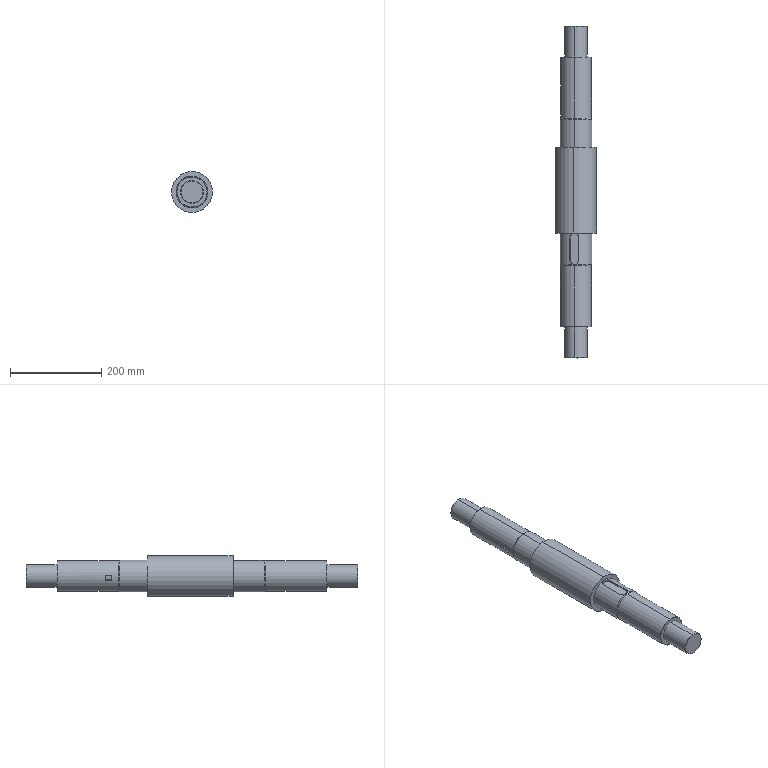Component | SolidWorks | LowerTensioningDeviceAssembly-1_LowerAxis-1 | 1 solid | 43 faces | volume 2952238 mm3 | cylinder 17 | plane 14 | cone 8 | torus 4 | commonest cylinder face diameters 50 x4 70 x4 68 x4 20 x3 90 x2